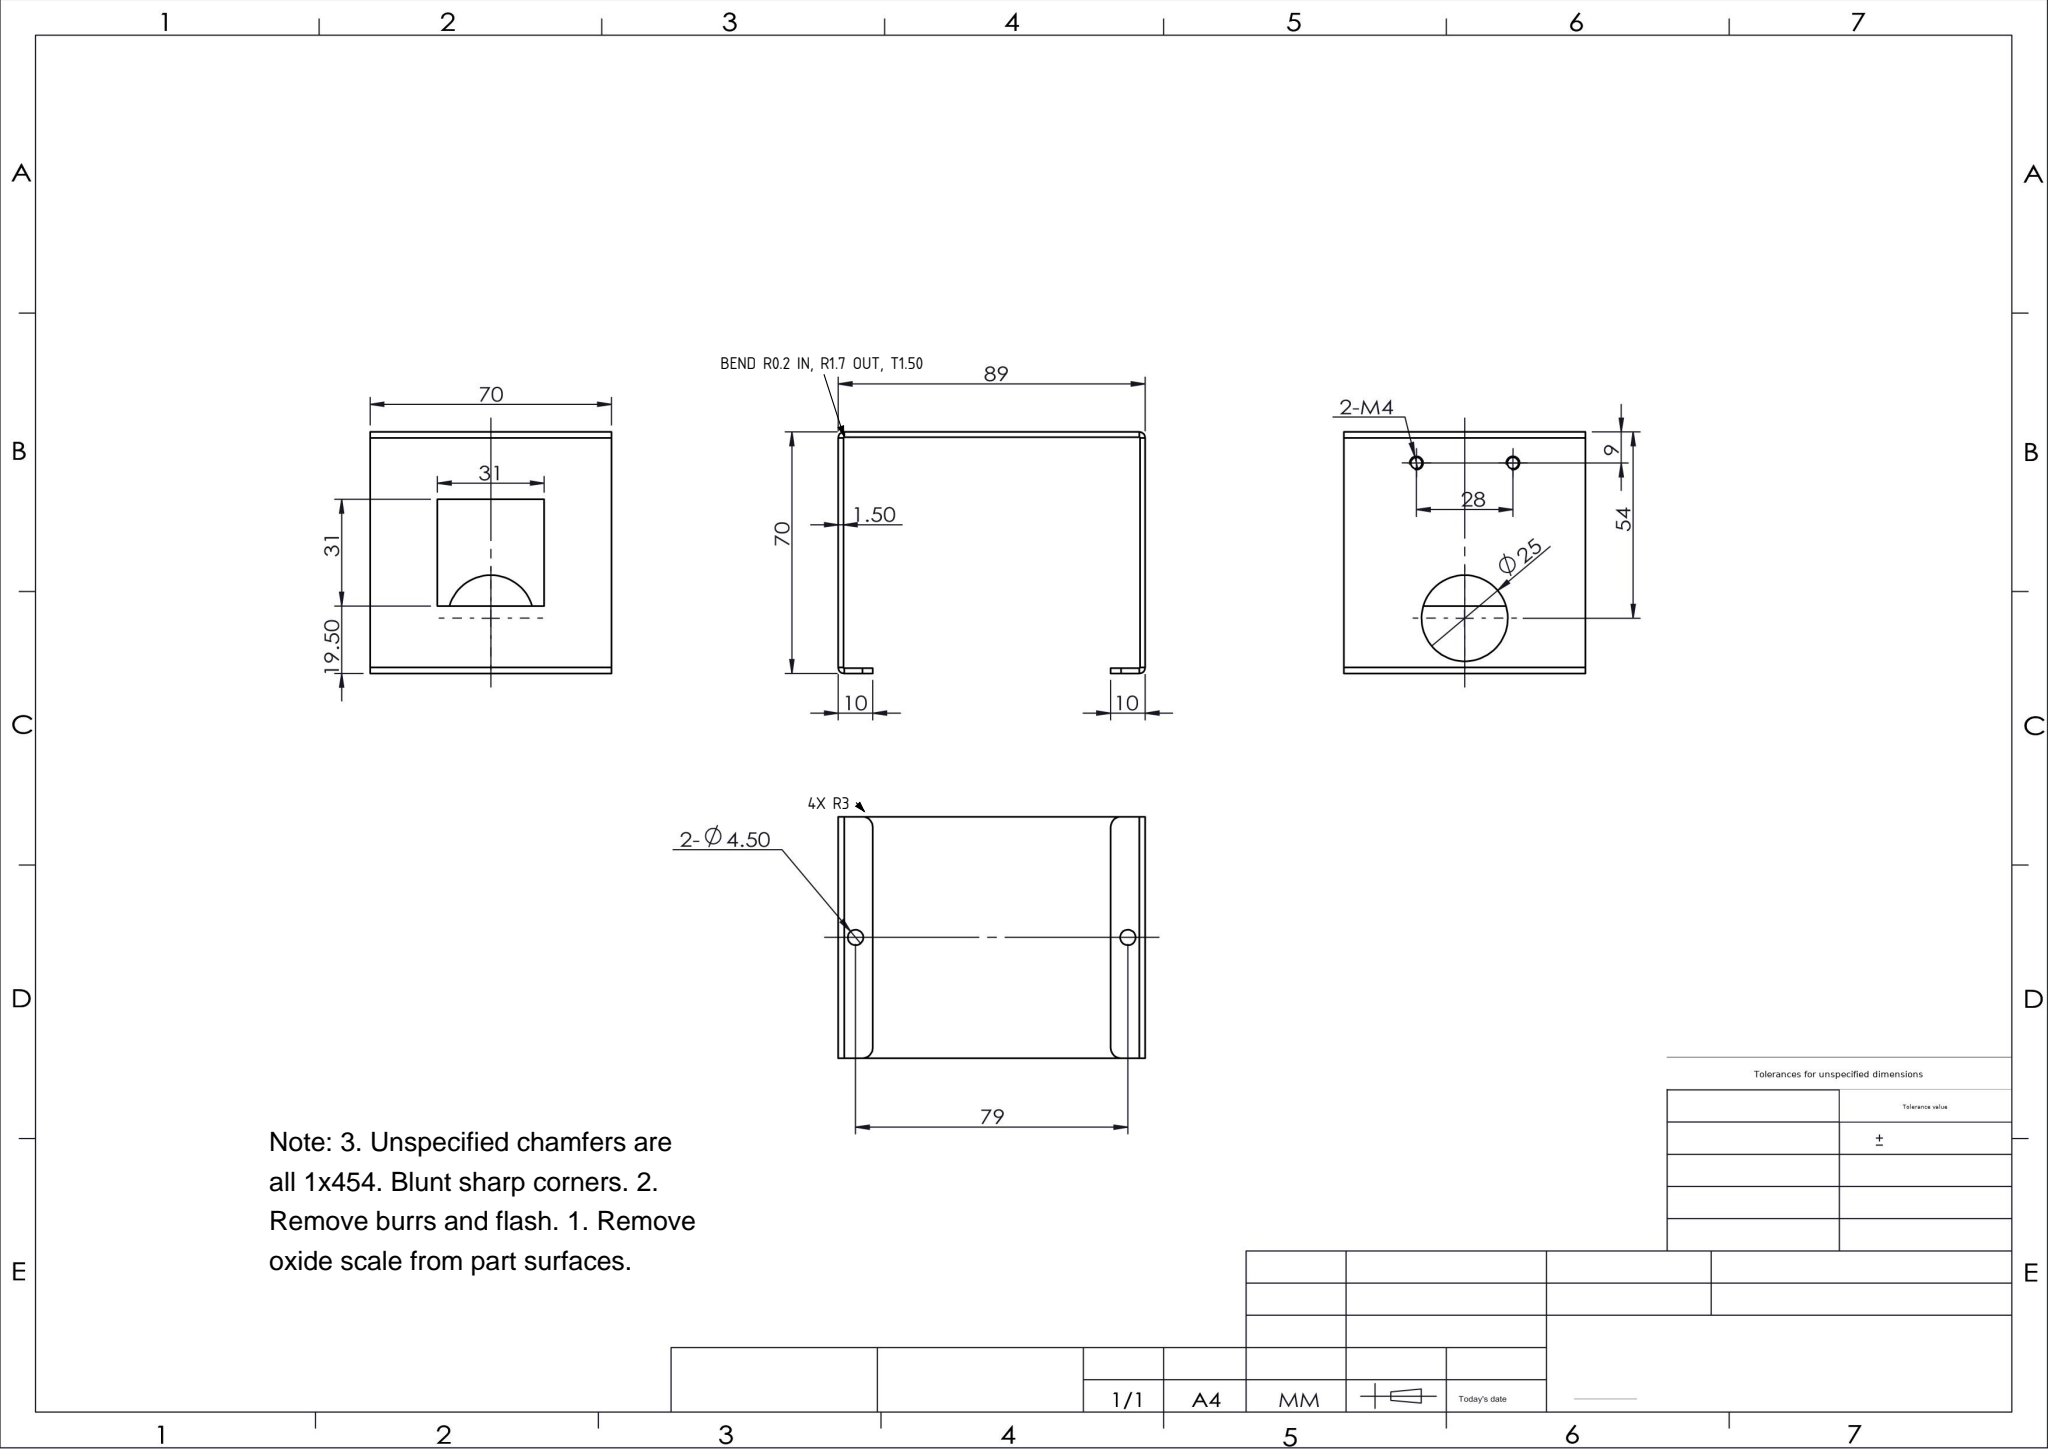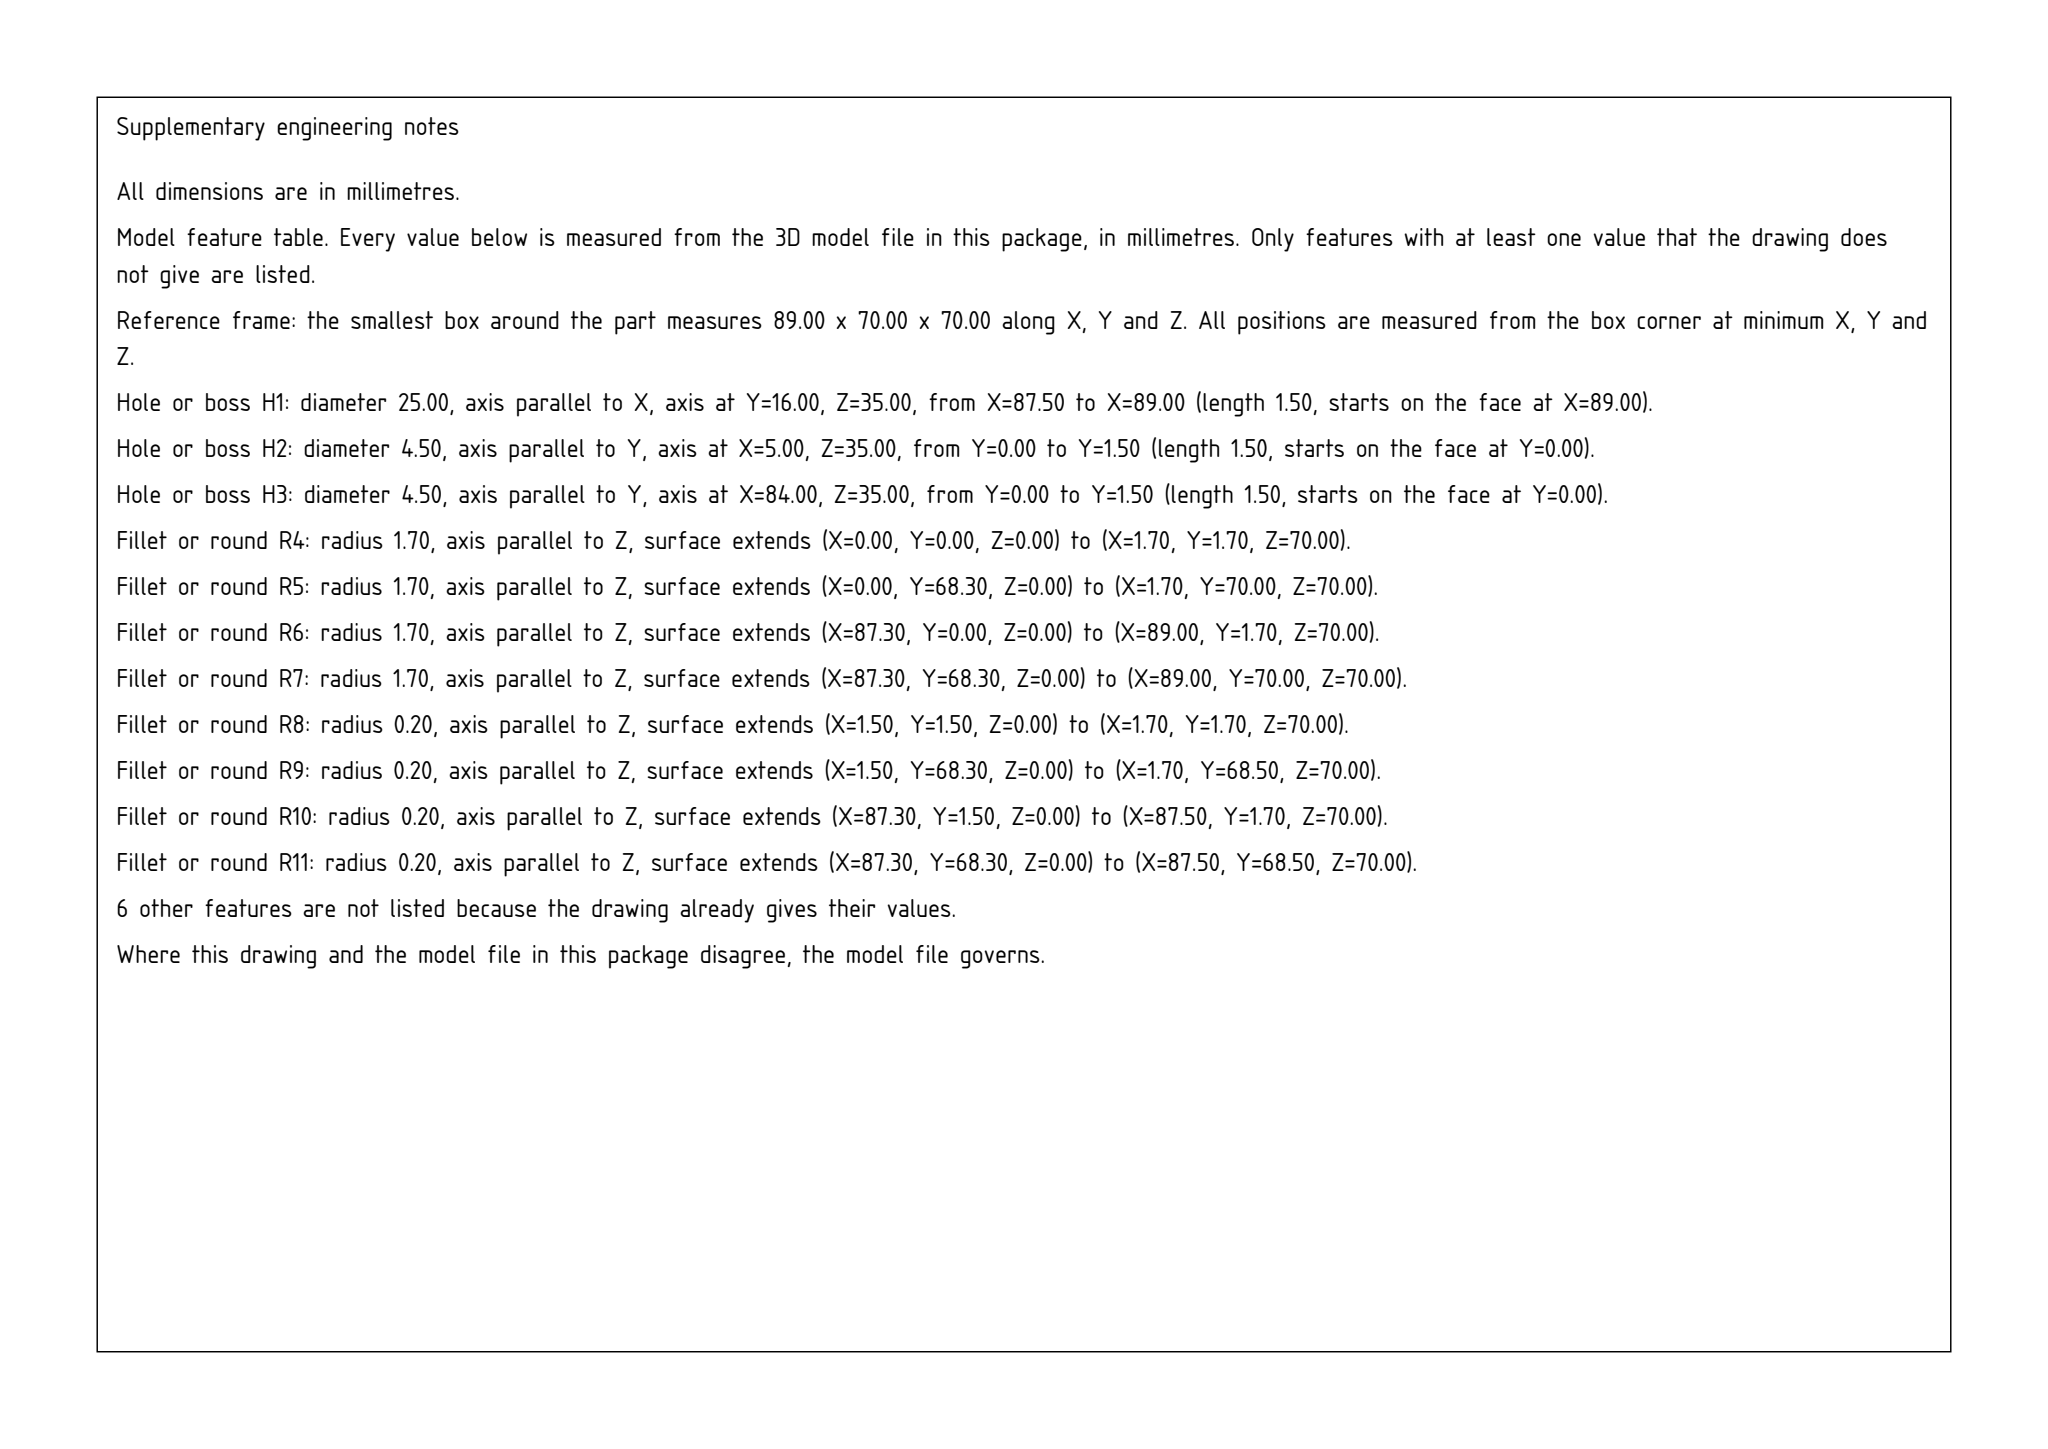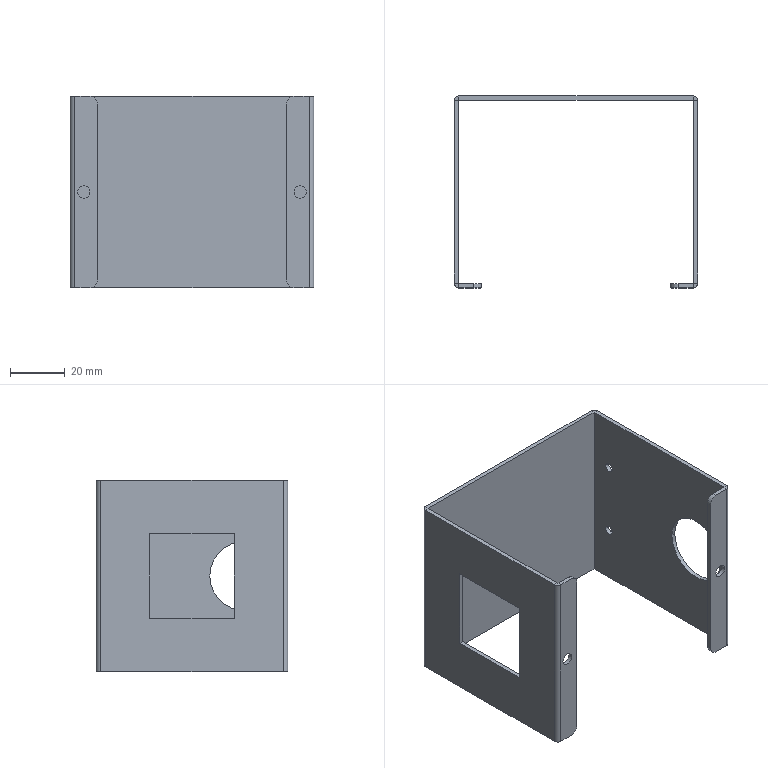Part | SolidWorks | mm | 1 solid | 56 faces | box 89 x 70 x 70 mm | volume 23081 mm3 | plane 34 | cylinder 22 | commonest cylinder face diameters 4.5 x4 3.3 x4 3.4 x4 0.4 x4 6 x4 25 x2
Drawing notes:
NOTE 3: UNSPECIFIED CHAMFERS 1X45 (C1); BLUNT SHARP CORNERS | from the solid: inclined_planes (chamfers/angled faces): none in STEP; only edge-break chamfers implied, note text restated as 1x45 deg (C1) per scrambled '1x454.' = '1x45' + note '4.'
ALL 4 BENDS: INNER R0.2, OUTER R1.7, THK 1.50 | from the solid: concave arcs dia 0.4 (R0.2) and convex arcs dia 3.4 (R1.7) at [1.7,1.7],[1.7,68.3],[87.3,1.7],[87.3,68.3], z0-70; wall 1.5
BOTTOM VIEW: R3 AT 4 CORNERS OF BOTTOM RETURN FLANGES | from the solid: convex arcs dia 6.0 about y at x=7 & 82, z=3 & 67, y from 0 to 1.5 (flange thk)